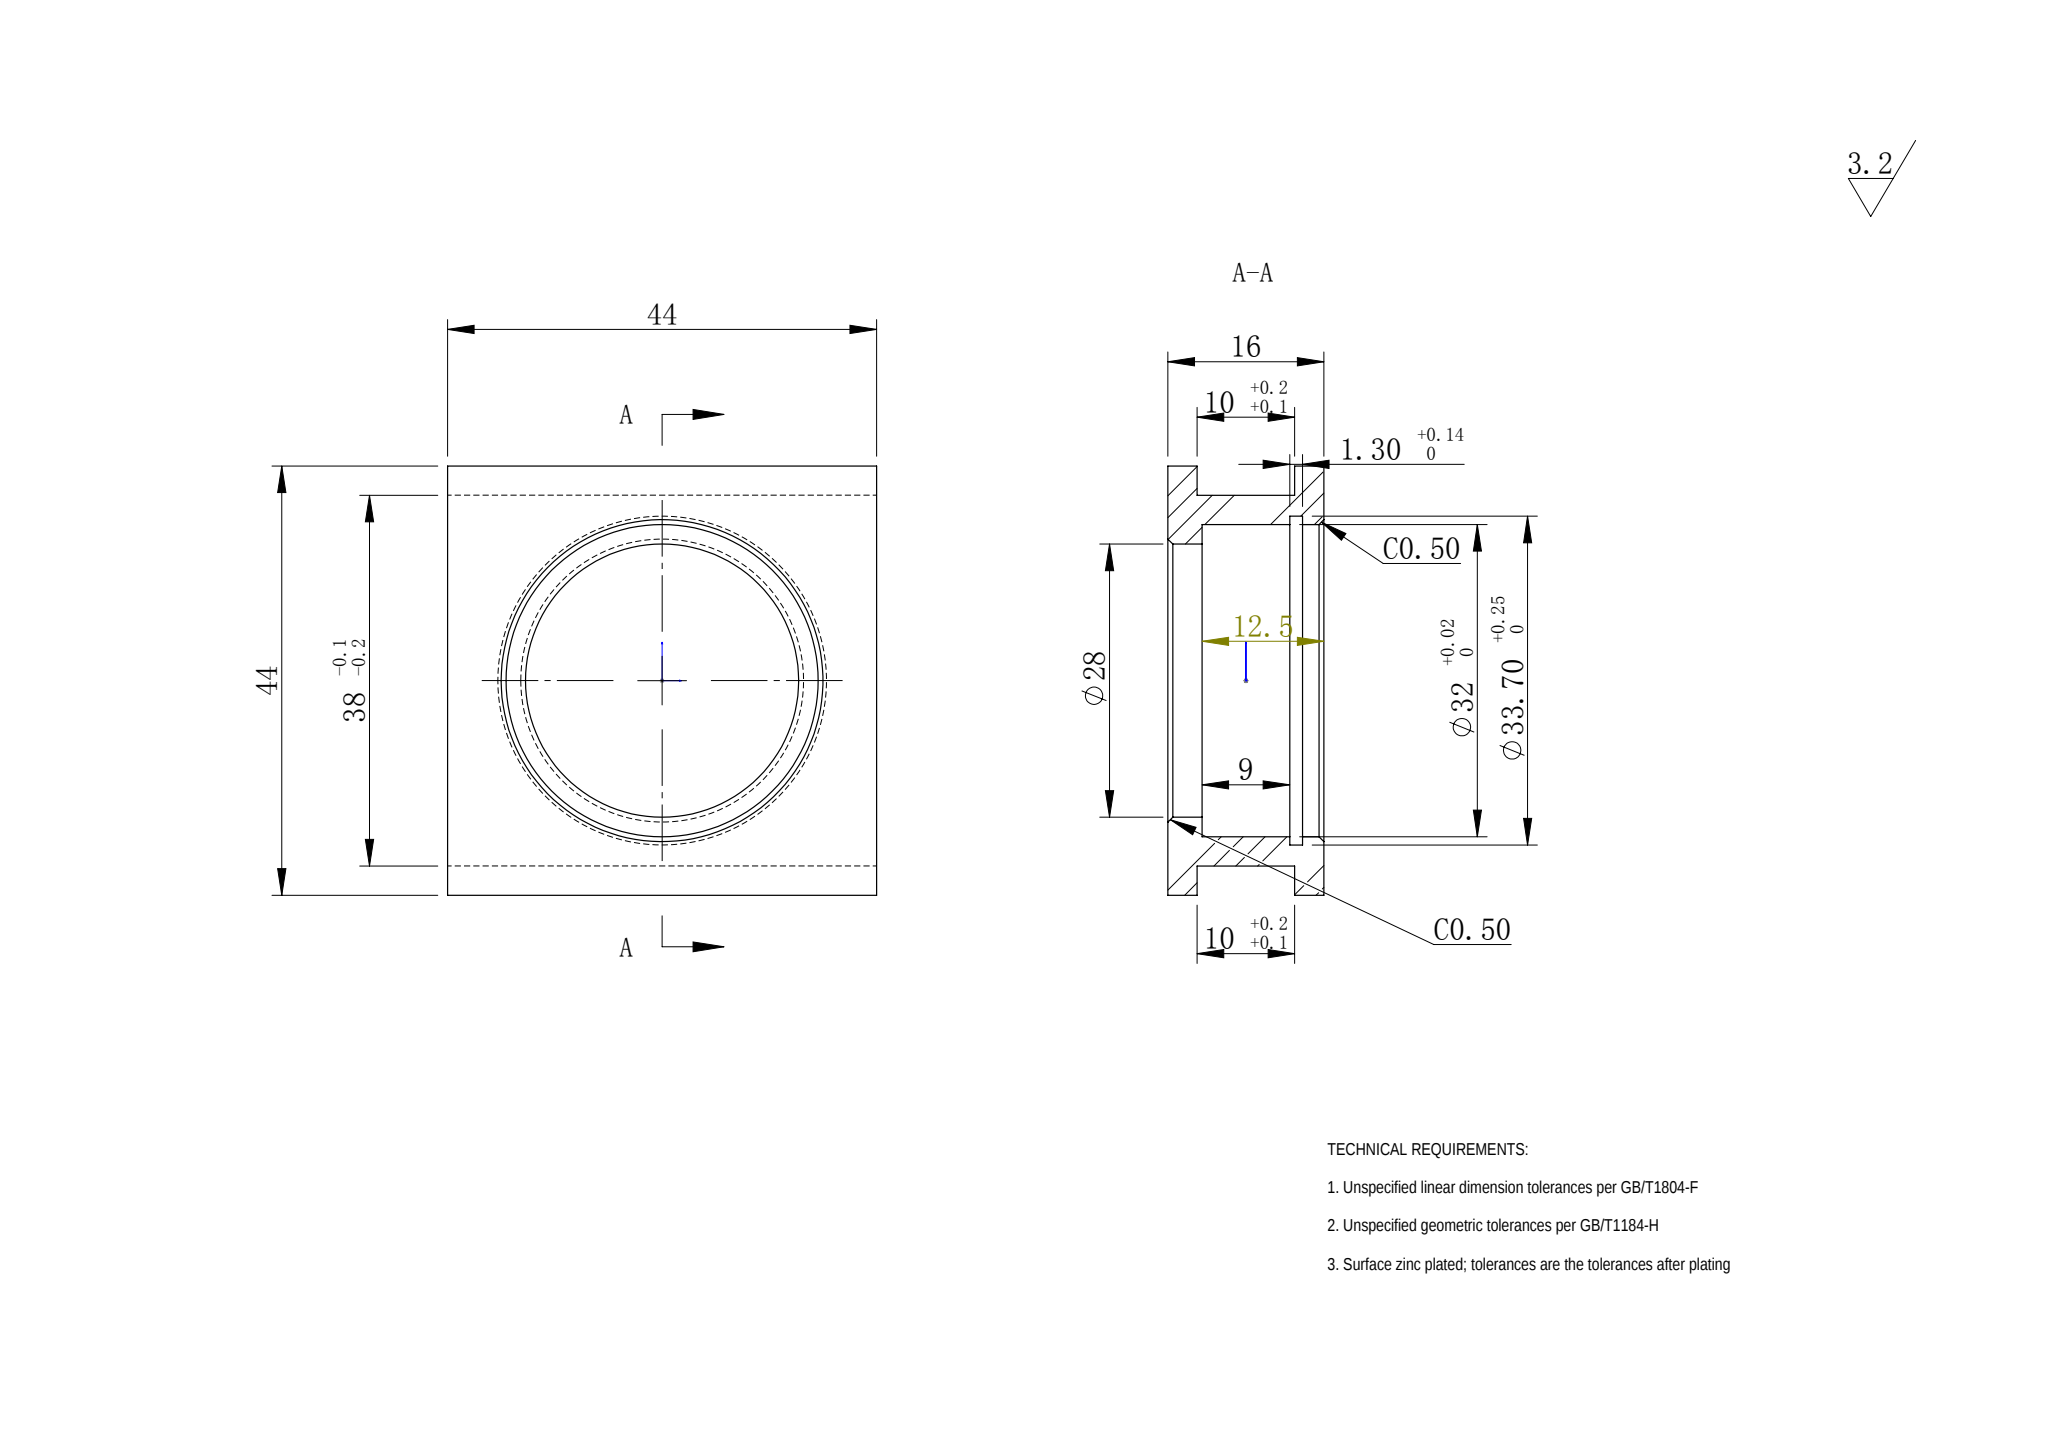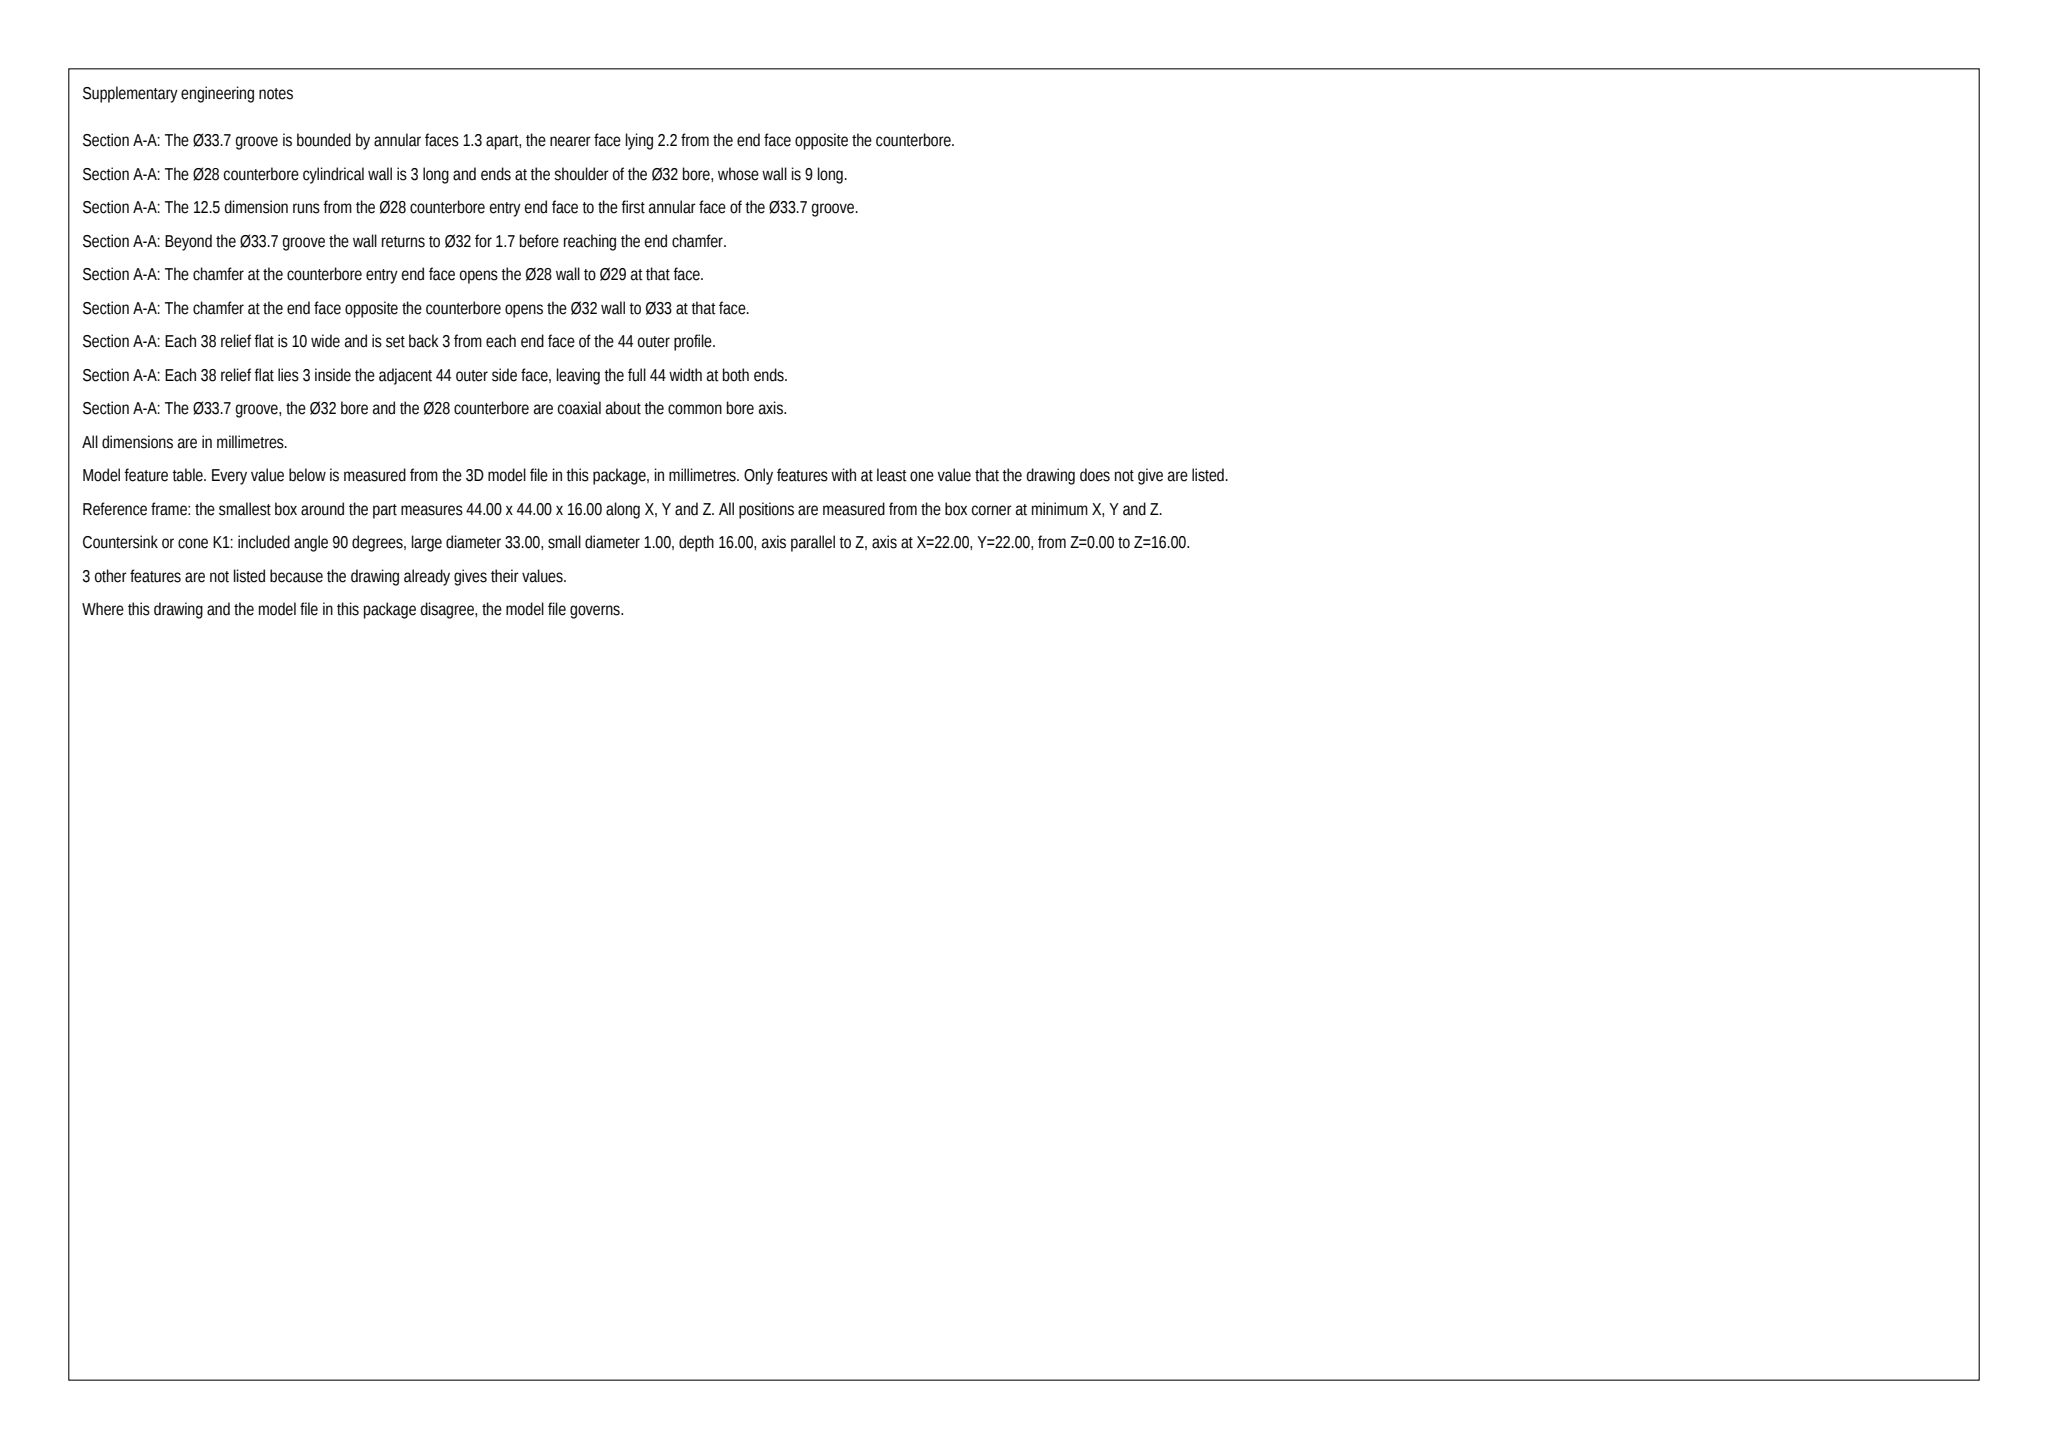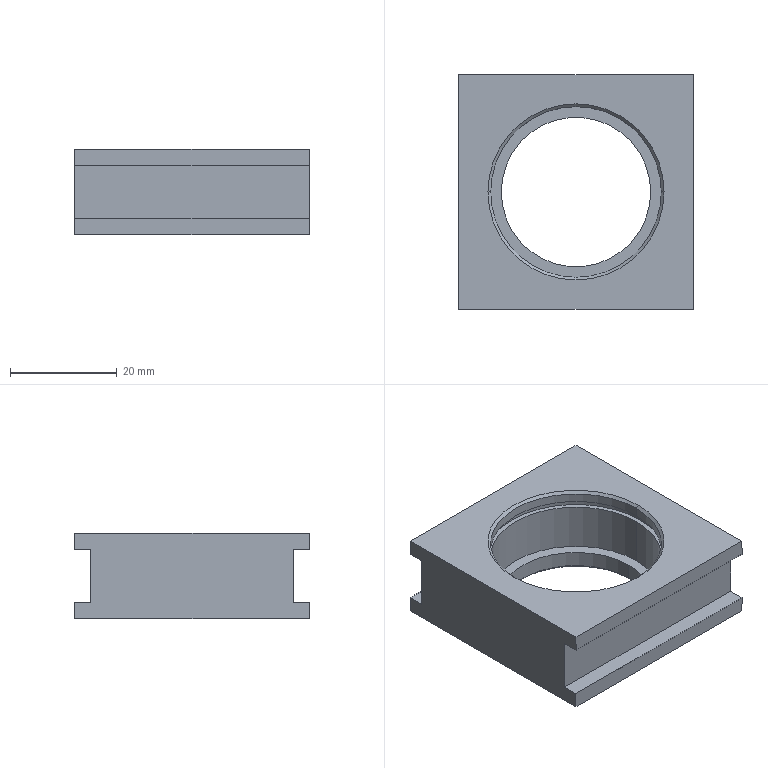Part | SolidWorks | mm | 1 solid | 29 faces | box 44 x 44 x 16 mm | volume 15990 mm3 | plane 17 | cylinder 8 | cone 4 | commonest cylinder face diameters 32 x4 33.7 x2 28 x2
build123d program:
from build123d import *

# Parameters (mm, degrees)
SKETCH1_W           = 44
SKETCH1_H           = 44
BOSS_EXTRUDE1_DEPTH = 8
SKETCH2_R           = 16
CUT_EXTRUDE1_DEPTH  = 12.5
SKETCH3_R           = 14
CUT_EXTRUDE2_DEPTH  = 34.53
SKETCH5_W           = 1.3
SKETCH5_H           = 0.85
SKETCH6_W           = 10
SKETCH6_H           = 3
CUT_EXTRUDE3_DEPTH  = 50.84
CHAMFER1_SIZE       = 0.5


with BuildPart() as part:
    # Sketch1 → Boss-Extrude1 (new, symmetric)
    with BuildSketch(Plane.XY):
        Rectangle(SKETCH1_W, SKETCH1_H)
    extrude(amount=BOSS_EXTRUDE1_DEPTH, both=True)

    # Sketch2 → Cut-Extrude1 (cut)
    with BuildSketch(Plane.XY.offset(8)):
        Circle(SKETCH2_R)
    extrude(amount=-CUT_EXTRUDE1_DEPTH, mode=Mode.SUBTRACT)

    # Sketch3 → Cut-Extrude2 (cut, through all)
    with BuildSketch(Plane.XY.offset(-4.5)):
        Circle(SKETCH3_R)
    extrude(amount=-CUT_EXTRUDE2_DEPTH, mode=Mode.SUBTRACT)

    # Sketch5 → Cut-Revolve1 (revolve, cut)
    with BuildSketch(Plane(origin=(0, 0, 0), x_dir=(0, 0, -1), z_dir=(1, 0, 0)), mode=Mode.PRIVATE) as cut_revolve1_sk:
        with Locations((-5.15, 16.425)):
            Rectangle(SKETCH5_W, SKETCH5_H)
    revolve(cut_revolve1_sk.sketch.rotate(Axis((0, 0, -9.603), (0, 0, 1)), 270), axis=Axis((0, 0, -9.603), (0, 0, 1)), mode=Mode.SUBTRACT)

    # Sketch6 → Cut-Extrude3 (cut, through all)
    with BuildSketch(Plane(origin=(22, 0, 0), x_dir=(0, 0, -1), z_dir=(1, 0, 0))):
        with Locations((0, 20.5)):
            Rectangle(SKETCH6_W, SKETCH6_H)
        with Locations((0, -20.5)):
            Rectangle(SKETCH6_W, SKETCH6_H)
    extrude(amount=-CUT_EXTRUDE3_DEPTH, mode=Mode.SUBTRACT)

    # Chamfer1
    chamfer1_edges = [part.edges().sort_by_distance(p)[0] for p in [
        (-16, 0, 8),
        (-14, 0, -8),
    ]]
    chamfer(chamfer1_edges, length=CHAMFER1_SIZE)


solid = part.part
STEP:
#1=CARTESIAN_POINT('',(-16.,0.,7.5));
#2=VERTEX_POINT('',#1);
#3=CARTESIAN_POINT('',(16.,0.,7.5));
#4=VERTEX_POINT('',#3);
#5=CARTESIAN_POINT('',(0.,0.,7.5));
#6=DIRECTION('',(0.,0.,1.));
#7=DIRECTION('',(-1.,0.,0.));
#8=AXIS2_PLACEMENT_3D('',#5,#6,#7);
#9=CIRCLE('',#8,16.);
#10=EDGE_CURVE('',#2,#4,#9,.T.);
#11=ORIENTED_EDGE('',*,*,#10,.F.);
#12=CARTESIAN_POINT('',(-16.5,0.,8.));
#13=VERTEX_POINT('',#12);
#14=CARTESIAN_POINT('',(-16.,0.,7.5));
#15=DIRECTION('',(-0.7071,0.,0.7071));
#16=VECTOR('',#15,1000.);
#17=LINE('',#14,#16);
#18=EDGE_CURVE('',#2,#13,#17,.T.);
#19=ORIENTED_EDGE('',*,*,#18,.T.);
#20=CARTESIAN_POINT('',(16.5,0.,8.));
#21=VERTEX_POINT('',#20);
#22=CARTESIAN_POINT('',(0.,0.,8.));
#23=DIRECTION('',(0.,0.,-1.));
#24=DIRECTION('',(-1.,0.,0.));
#25=AXIS2_PLACEMENT_3D('',#22,#23,#24);
#26=CIRCLE('',#25,16.5);
#27=EDGE_CURVE('',#21,#13,#26,.T.);
#28=ORIENTED_EDGE('',*,*,#27,.F.);
#29=CARTESIAN_POINT('',(16.,0.,7.5));
#30=DIRECTION('',(0.7071,0.,0.7071));
#31=VECTOR('',#30,1000.);
#32=LINE('',#29,#31);
#33=EDGE_CURVE('',#4,#21,#32,.T.);
#34=ORIENTED_EDGE('',*,*,#33,.F.);
#35=EDGE_LOOP('',(#11,#19,#28,#34));
#36=FACE_OUTER_BOUND('',#35,.T.);
#37=CARTESIAN_POINT('',(0.,0.,7.5));
#38=DIRECTION('',(0.,0.,1.));
#39=DIRECTION('',(1.,0.,0.));
#40=AXIS2_PLACEMENT_3D('',#37,#38,#39);
#41=CONICAL_SURFACE('',#40,16.,0.7854);
#42=ADVANCED_FACE('',(#36),#41,.F.);
#43=CARTESIAN_POINT('',(14.,0.,-7.5));
#44=VERTEX_POINT('',#43);
#45=CARTESIAN_POINT('',(-14.,0.,-7.5));
#46=VERTEX_POINT('',#45);
#47=CARTESIAN_POINT('',(0.,0.,-7.5));
#48=DIRECTION('',(0.,0.,-1.));
#49=DIRECTION('',(-1.,0.,0.));
#50=AXIS2_PLACEMENT_3D('',#47,#48,#49);
#51=CIRCLE('',#50,14.);
#52=EDGE_CURVE('',#44,#46,#51,.T.);
#53=ORIENTED_EDGE('',*,*,#52,.F.);
#54=CARTESIAN_POINT('',(14.5,0.,-8.));
#55=VERTEX_POINT('',#54);
#56=CARTESIAN_POINT('',(14.5,0.,-8.));
#57=DIRECTION('',(0.7071,0.,-0.7071));
#58=VECTOR('',#57,1000.);
#59=LINE('',#56,#58);
#60=EDGE_CURVE('',#44,#55,#59,.T.);
#61=ORIENTED_EDGE('',*,*,#60,.T.);
#62=CARTESIAN_POINT('',(-14.5,0.,-8.));
#63=VERTEX_POINT('',#62);
#64=CARTESIAN_POINT('',(0.,0.,-8.));
#65=DIRECTION('',(0.,0.,1.));
#66=DIRECTION('',(-1.,0.,0.));
#67=AXIS2_PLACEMENT_3D('',#64,#65,#66);
#68=CIRCLE('',#67,14.5);
#69=EDGE_CURVE('',#63,#55,#68,.T.);
#70=ORIENTED_EDGE('',*,*,#69,.F.);
#71=CARTESIAN_POINT('',(-14.5,0.,-8.));
#72=DIRECTION('',(-0.7071,0.,-0.7071));
#73=VECTOR('',#72,1000.);
#74=LINE('',#71,#73);
#75=EDGE_CURVE('',#46,#63,#74,.T.);
#76=ORIENTED_EDGE('',*,*,#75,.F.);
#77=EDGE_LOOP('',(#53,#61,#70,#76));
#78=FACE_OUTER_BOUND('',#77,.T.);
#79=CARTESIAN_POINT('',(0.,0.,-8.));
#80=DIRECTION('',(0.,0.,-1.));
#81=DIRECTION('',(-1.,0.,0.));
#82=AXIS2_PLACEMENT_3D('',#79,#80,#81);
#83=CONICAL_SURFACE('',#82,14.5,0.7854);
#84=ADVANCED_FACE('',(#78),#83,.F.);
#85=CARTESIAN_POINT('',(16.85,0.,5.8));
#86=VERTEX_POINT('',#85);
#87=CARTESIAN_POINT('',(-16.85,0.,5.8));
#88=VERTEX_POINT('',#87);
#89=CARTESIAN_POINT('',(0.,0.,5.8));
#90=DIRECTION('',(0.,0.,-1.));
#91=DIRECTION('',(-1.,0.,0.));
#92=AXIS2_PLACEMENT_3D('',#89,#90,#91);
#93=CIRCLE('',#92,16.85);
#94=EDGE_CURVE('',#86,#88,#93,.T.);
#95=ORIENTED_EDGE('',*,*,#94,.F.);
#96=CARTESIAN_POINT('',(16.85,0.,4.5));
#97=VERTEX_POINT('',#96);
#98=CARTESIAN_POINT('',(16.85,0.,-9.603));
#99=DIRECTION('',(0.,0.,-1.));
#100=VECTOR('',#99,1000.);
#101=LINE('',#98,#100);
#102=EDGE_CURVE('',#86,#97,#101,.T.);
#103=ORIENTED_EDGE('',*,*,#102,.T.);
#104=CARTESIAN_POINT('',(-16.85,0.,4.5));
#105=VERTEX_POINT('',#104);
#106=CARTESIAN_POINT('',(0.,0.,4.5));
#107=DIRECTION('',(0.,0.,-1.));
#108=DIRECTION('',(-1.,0.,0.));
#109=AXIS2_PLACEMENT_3D('',#106,#107,#108);
#110=CIRCLE('',#109,16.85);
#111=EDGE_CURVE('',#97,#105,#110,.T.);
#112=ORIENTED_EDGE('',*,*,#111,.T.);
#113=CARTESIAN_POINT('',(-16.85,0.,-9.603));
#114=DIRECTION('',(0.,0.,-1.));
#115=VECTOR('',#114,1000.);
#116=LINE('',#113,#115);
#117=EDGE_CURVE('',#88,#105,#116,.T.);
#118=ORIENTED_EDGE('',*,*,#117,.F.);
#119=EDGE_LOOP('',(#95,#103,#112,#118));
#120=FACE_OUTER_BOUND('',#119,.T.);
#121=CARTESIAN_POINT('',(0.,0.,-9.603));
#122=DIRECTION('',(0.,0.,-1.));
#123=DIRECTION('',(-1.,0.,0.));
#124=AXIS2_PLACEMENT_3D('',#121,#122,#123);
#125=CYLINDRICAL_SURFACE('',#124,16.85);
#126=ADVANCED_FACE('',(#120),#125,.F.);
#127=ORIENTED_EDGE('',*,*,#52,.T.);
#128=CARTESIAN_POINT('',(-14.,0.,-4.5));
#129=VERTEX_POINT('',#128);
#130=CARTESIAN_POINT('',(-14.,0.,-8.));
#131=DIRECTION('',(0.,0.,1.));
#132=VECTOR('',#131,1000.);
#133=LINE('',#130,#132);
#134=EDGE_CURVE('',#46,#129,#133,.T.);
#135=ORIENTED_EDGE('',*,*,#134,.T.);
#136=CARTESIAN_POINT('',(14.,0.,-4.5));
#137=VERTEX_POINT('',#136);
#138=CARTESIAN_POINT('',(0.,0.,-4.5));
#139=DIRECTION('',(0.,0.,1.));
#140=DIRECTION('',(1.,0.,0.));
#141=AXIS2_PLACEMENT_3D('',#138,#139,#140);
#142=CIRCLE('',#141,14.);
#143=EDGE_CURVE('',#129,#137,#142,.T.);
#144=ORIENTED_EDGE('',*,*,#143,.T.);
#145=CARTESIAN_POINT('',(14.,0.,-8.));
#146=DIRECTION('',(0.,0.,1.));
#147=VECTOR('',#146,1000.);
#148=LINE('',#145,#147);
#149=EDGE_CURVE('',#44,#137,#148,.T.);
#150=ORIENTED_EDGE('',*,*,#149,.F.);
#151=EDGE_LOOP('',(#127,#135,#144,#150));
#152=FACE_OUTER_BOUND('',#151,.T.);
#153=CARTESIAN_POINT('',(0.,0.,-8.));
#154=DIRECTION('',(0.,0.,1.));
#155=DIRECTION('',(1.,0.,0.));
#156=AXIS2_PLACEMENT_3D('',#153,#154,#155);
#157=CYLINDRICAL_SURFACE('',#156,14.);
#158=ADVANCED_FACE('',(#152),#157,.F.);
#159=CARTESIAN_POINT('',(16.,0.,5.8));
#160=VERTEX_POINT('',#159);
#161=CARTESIAN_POINT('',(-16.,0.,5.8));
#162=VERTEX_POINT('',#161);
#163=CARTESIAN_POINT('',(0.,0.,5.8));
#164=DIRECTION('',(0.,0.,-1.));
#165=DIRECTION('',(-1.,0.,0.));
#166=AXIS2_PLACEMENT_3D('',#163,#164,#165);
#167=CIRCLE('',#166,16.);
#168=EDGE_CURVE('',#160,#162,#167,.T.);
#169=ORIENTED_EDGE('',*,*,#168,.T.);
#170=CARTESIAN_POINT('',(-16.,0.,-4.5));
#171=DIRECTION('',(0.,0.,1.));
#172=VECTOR('',#171,1000.);
#173=LINE('',#170,#172);
#174=EDGE_CURVE('',#162,#2,#173,.T.);
#175=ORIENTED_EDGE('',*,*,#174,.T.);
#176=ORIENTED_EDGE('',*,*,#10,.T.);
#177=CARTESIAN_POINT('',(16.,0.,-4.5));
#178=DIRECTION('',(0.,0.,1.));
#179=VECTOR('',#178,1000.);
#180=LINE('',#177,#179);
#181=EDGE_CURVE('',#160,#4,#180,.T.);
#182=ORIENTED_EDGE('',*,*,#181,.F.);
#183=EDGE_LOOP('',(#169,#175,#176,#182));
#184=FACE_OUTER_BOUND('',#183,.T.);
#185=CARTESIAN_POINT('',(0.,0.,-4.5));
#186=DIRECTION('',(0.,0.,1.));
#187=DIRECTION('',(1.,0.,0.));
#188=AXIS2_PLACEMENT_3D('',#185,#186,#187);
#189=CYLINDRICAL_SURFACE('',#188,16.);
#190=ADVANCED_FACE('',(#184),#189,.F.);
#191=CARTESIAN_POINT('',(-16.,0.,-4.5));
#192=VERTEX_POINT('',#191);
#193=CARTESIAN_POINT('',(16.,0.,-4.5));
#194=VERTEX_POINT('',#193);
#195=CARTESIAN_POINT('',(0.,0.,-4.5));
#196=DIRECTION('',(0.,0.,1.));
#197=DIRECTION('',(1.,0.,0.));
#198=AXIS2_PLACEMENT_3D('',#195,#196,#197);
#199=CIRCLE('',#198,16.);
#200=EDGE_CURVE('',#192,#194,#199,.T.);
#201=ORIENTED_EDGE('',*,*,#200,.F.);
#202=CARTESIAN_POINT('',(-16.,0.,4.5));
#203=VERTEX_POINT('',#202);
#204=CARTESIAN_POINT('',(-16.,0.,-4.5));
#205=DIRECTION('',(0.,0.,1.));
#206=VECTOR('',#205,1000.);
#207=LINE('',#204,#206);
#208=EDGE_CURVE('',#192,#203,#207,.T.);
#209=ORIENTED_EDGE('',*,*,#208,.T.);
#210=CARTESIAN_POINT('',(16.,0.,4.5));
#211=VERTEX_POINT('',#210);
#212=CARTESIAN_POINT('',(0.,0.,4.5));
#213=DIRECTION('',(0.,0.,-1.));
#214=DIRECTION('',(-1.,0.,0.));
#215=AXIS2_PLACEMENT_3D('',#212,#213,#214);
#216=CIRCLE('',#215,16.);
#217=EDGE_CURVE('',#211,#203,#216,.T.);
#218=ORIENTED_EDGE('',*,*,#217,.F.);
#219=CARTESIAN_POINT('',(16.,0.,-4.5));
#220=DIRECTION('',(0.,0.,1.));
#221=VECTOR('',#220,1000.);
#222=LINE('',#219,#221);
#223=EDGE_CURVE('',#194,#211,#222,.T.);
#224=ORIENTED_EDGE('',*,*,#223,.F.);
#225=EDGE_LOOP('',(#201,#209,#218,#224));
#226=FACE_OUTER_BOUND('',#225,.T.);
#227=CARTESIAN_POINT('',(0.,0.,-4.5));
#228=DIRECTION('',(0.,0.,1.));
#229=DIRECTION('',(1.,0.,0.));
#230=AXIS2_PLACEMENT_3D('',#227,#228,#229);
#231=CYLINDRICAL_SURFACE('',#230,16.);
#232=ADVANCED_FACE('',(#226),#231,.F.);
#233=CARTESIAN_POINT('',(-22.,-22.,8.));
#234=VERTEX_POINT('',#233);
#235=CARTESIAN_POINT('',(-22.,-22.,5.));
#236=VERTEX_POINT('',#235);
#237=CARTESIAN_POINT('',(-22.,-22.,8.));
#238=DIRECTION('',(0.,0.,-1.));
#239=VECTOR('',#238,1000.);
#240=LINE('',#237,#239);
#241=EDGE_CURVE('',#234,#236,#240,.T.);
#242=ORIENTED_EDGE('',*,*,#241,.T.);
#243=CARTESIAN_POINT('',(22.,-22.,5.));
#244=VERTEX_POINT('',#243);
#245=CARTESIAN_POINT('',(-22.,-22.,5.));
#246=DIRECTION('',(1.,0.,0.));
#247=VECTOR('',#246,1000.);
#248=LINE('',#245,#247);
#249=EDGE_CURVE('',#236,#244,#248,.T.);
#250=ORIENTED_EDGE('',*,*,#249,.T.);
#251=CARTESIAN_POINT('',(22.,-22.,8.));
#252=VERTEX_POINT('',#251);
#253=CARTESIAN_POINT('',(22.,-22.,8.));
#254=DIRECTION('',(0.,0.,-1.));
#255=VECTOR('',#254,1000.);
#256=LINE('',#253,#255);
#257=EDGE_CURVE('',#252,#244,#256,.T.);
#258=ORIENTED_EDGE('',*,*,#257,.F.);
#259=CARTESIAN_POINT('',(-22.,-22.,8.));
#260=DIRECTION('',(1.,0.,0.));
#261=VECTOR('',#260,1000.);
#262=LINE('',#259,#261);
#263=EDGE_CURVE('',#234,#252,#262,.T.);
#264=ORIENTED_EDGE('',*,*,#263,.F.);
#265=EDGE_LOOP('',(#242,#250,#258,#264));
#266=FACE_OUTER_BOUND('',#265,.T.);
#267=CARTESIAN_POINT('',(-22.,-22.,8.));
#268=DIRECTION('',(0.,1.,0.));
#269=DIRECTION('',(0.,0.,1.));
#270=AXIS2_PLACEMENT_3D('',#267,#268,#269);
#271=PLANE('',#270);
#272=ADVANCED_FACE('',(#266),#271,.F.);
#273=CARTESIAN_POINT('',(22.,22.,8.));
#274=VERTEX_POINT('',#273);
#275=CARTESIAN_POINT('',(22.,22.,5.));
#276=VERTEX_POINT('',#275);
#277=CARTESIAN_POINT('',(22.,22.,8.));
#278=DIRECTION('',(0.,0.,-1.));
#279=VECTOR('',#278,1000.);
#280=LINE('',#277,#279);
#281=EDGE_CURVE('',#274,#276,#280,.T.);
#282=ORIENTED_EDGE('',*,*,#281,.T.);
#283=CARTESIAN_POINT('',(-22.,22.,5.));
#284=VERTEX_POINT('',#283);
#285=CARTESIAN_POINT('',(-22.,22.,5.));
#286=DIRECTION('',(1.,0.,0.));
#287=VECTOR('',#286,1000.);
#288=LINE('',#285,#287);
#289=EDGE_CURVE('',#284,#276,#288,.T.);
#290=ORIENTED_EDGE('',*,*,#289,.F.);
#291=CARTESIAN_POINT('',(-22.,22.,8.));
#292=VERTEX_POINT('',#291);
#293=CARTESIAN_POINT('',(-22.,22.,8.));
#294=DIRECTION('',(0.,0.,-1.));
#295=VECTOR('',#294,1000.);
#296=LINE('',#293,#295);
#297=EDGE_CURVE('',#292,#284,#296,.T.);
#298=ORIENTED_EDGE('',*,*,#297,.F.);
#299=CARTESIAN_POINT('',(-22.,22.,8.));
#300=DIRECTION('',(-1.,0.,0.));
#301=VECTOR('',#300,1000.);
#302=LINE('',#299,#301);
#303=EDGE_CURVE('',#274,#292,#302,.T.);
#304=ORIENTED_EDGE('',*,*,#303,.F.);
#305=EDGE_LOOP('',(#282,#290,#298,#304));
#306=FACE_OUTER_BOUND('',#305,.T.);
#307=CARTESIAN_POINT('',(-22.,22.,8.));
#308=DIRECTION('',(0.,-1.,0.));
#309=DIRECTION('',(0.,0.,-1.));
#310=AXIS2_PLACEMENT_3D('',#307,#308,#309);
#311=PLANE('',#310);
#312=ADVANCED_FACE('',(#306),#311,.F.);
#313=ORIENTED_EDGE('',*,*,#208,.F.);
#314=CARTESIAN_POINT('',(0.,0.,-4.5));
#315=DIRECTION('',(0.,0.,1.));
#316=DIRECTION('',(1.,0.,0.));
#317=AXIS2_PLACEMENT_3D('',#314,#315,#316);
#318=CIRCLE('',#317,16.);
#319=EDGE_CURVE('',#194,#192,#318,.T.);
#320=ORIENTED_EDGE('',*,*,#319,.F.);
#321=ORIENTED_EDGE('',*,*,#223,.T.);
#322=CARTESIAN_POINT('',(0.,0.,4.5));
#323=DIRECTION('',(0.,0.,-1.));
#324=DIRECTION('',(-1.,0.,0.));
#325=AXIS2_PLACEMENT_3D('',#322,#323,#324);
#326=CIRCLE('',#325,16.);
#327=EDGE_CURVE('',#203,#211,#326,.T.);
#328=ORIENTED_EDGE('',*,*,#327,.F.);
#329=EDGE_LOOP('',(#313,#320,#321,#328));
#330=FACE_OUTER_BOUND('',#329,.T.);
#331=CARTESIAN_POINT('',(0.,0.,-4.5));
#332=DIRECTION('',(0.,0.,1.));
#333=DIRECTION('',(1.,0.,0.));
#334=AXIS2_PLACEMENT_3D('',#331,#332,#333);
#335=CYLINDRICAL_SURFACE('',#334,16.);
#336=ADVANCED_FACE('',(#330),#335,.F.);
#337=ORIENTED_EDGE('',*,*,#257,.T.);
#338=CARTESIAN_POINT('',(22.,-19.,5.));
#339=VERTEX_POINT('',#338);
#340=CARTESIAN_POINT('',(22.,-22.,5.));
#341=DIRECTION('',(0.,-1.,-0.));
#342=VECTOR('',#341,1000.);
#343=LINE('',#340,#342);
#344=EDGE_CURVE('',#339,#244,#343,.T.);
#345=ORIENTED_EDGE('',*,*,#344,.F.);
#346=CARTESIAN_POINT('',(22.,-19.,-5.));
#347=VERTEX_POINT('',#346);
#348=CARTESIAN_POINT('',(22.,-19.,5.));
#349=DIRECTION('',(0.,0.,1.));
#350=VECTOR('',#349,1000.);
#351=LINE('',#348,#350);
#352=EDGE_CURVE('',#347,#339,#351,.T.);
#353=ORIENTED_EDGE('',*,*,#352,.F.);
#354=CARTESIAN_POINT('',(22.,-22.,-5.));
#355=VERTEX_POINT('',#354);
#356=CARTESIAN_POINT('',(22.,-22.,-5.));
#357=DIRECTION('',(0.,1.,-0.));
#358=VECTOR('',#357,1000.);
#359=LINE('',#356,#358);
#360=EDGE_CURVE('',#355,#347,#359,.T.);
#361=ORIENTED_EDGE('',*,*,#360,.F.);
#362=CARTESIAN_POINT('',(22.,-22.,-8.));
#363=VERTEX_POINT('',#362);
#364=CARTESIAN_POINT('',(22.,-22.,8.));
#365=DIRECTION('',(0.,0.,-1.));
#366=VECTOR('',#365,1000.);
#367=LINE('',#364,#366);
#368=EDGE_CURVE('',#355,#363,#367,.T.);
#369=ORIENTED_EDGE('',*,*,#368,.T.);
#370=CARTESIAN_POINT('',(22.,22.,-8.));
#371=VERTEX_POINT('',#370);
#372=CARTESIAN_POINT('',(22.,-22.,-8.));
#373=DIRECTION('',(0.,1.,0.));
#374=VECTOR('',#373,1000.);
#375=LINE('',#372,#374);
#376=EDGE_CURVE('',#363,#371,#375,.T.);
#377=ORIENTED_EDGE('',*,*,#376,.T.);
#378=CARTESIAN_POINT('',(22.,22.,-5.));
#379=VERTEX_POINT('',#378);
#380=CARTESIAN_POINT('',(22.,22.,8.));
#381=DIRECTION('',(0.,0.,-1.));
#382=VECTOR('',#381,1000.);
#383=LINE('',#380,#382);
#384=EDGE_CURVE('',#379,#371,#383,.T.);
#385=ORIENTED_EDGE('',*,*,#384,.F.);
#386=CARTESIAN_POINT('',(22.,19.,-5.));
#387=VERTEX_POINT('',#386);
#388=CARTESIAN_POINT('',(22.,22.,-5.));
#389=DIRECTION('',(0.,1.,0.));
#390=VECTOR('',#389,1000.);
#391=LINE('',#388,#390);
#392=EDGE_CURVE('',#387,#379,#391,.T.);
#393=ORIENTED_EDGE('',*,*,#392,.F.);
#394=CARTESIAN_POINT('',(22.,19.,5.));
#395=VERTEX_POINT('',#394);
#396=CARTESIAN_POINT('',(22.,19.,5.));
#397=DIRECTION('',(0.,0.,-1.));
#398=VECTOR('',#397,1000.);
#399=LINE('',#396,#398);
#400=EDGE_CURVE('',#395,#387,#399,.T.);
#401=ORIENTED_EDGE('',*,*,#400,.F.);
#402=CARTESIAN_POINT('',(22.,22.,5.));
#403=DIRECTION('',(0.,-1.,0.));
#404=VECTOR('',#403,1000.);
#405=LINE('',#402,#404);
#406=EDGE_CURVE('',#276,#395,#405,.T.);
#407=ORIENTED_EDGE('',*,*,#406,.F.);
#408=ORIENTED_EDGE('',*,*,#281,.F.);
#409=CARTESIAN_POINT('',(22.,-22.,8.));
#410=DIRECTION('',(0.,1.,0.));
#411=VECTOR('',#410,1000.);
#412=LINE('',#409,#411);
#413=EDGE_CURVE('',#252,#274,#412,.T.);
#414=ORIENTED_EDGE('',*,*,#413,.F.);
#415=EDGE_LOOP('',(#337,#345,#353,#361,#369,#377,#385,#393,#401,#407,#408,#414));
#416=FACE_OUTER_BOUND('',#415,.T.);
#417=CARTESIAN_POINT('',(22.,-22.,8.));
#418=DIRECTION('',(-1.,0.,0.));
#419=DIRECTION('',(0.,0.,1.));
#420=AXIS2_PLACEMENT_3D('',#417,#418,#419);
#421=PLANE('',#420);
#422=ADVANCED_FACE('',(#416),#421,.F.);
#423=CARTESIAN_POINT('',(-22.,22.,-5.));
#424=VERTEX_POINT('',#423);
#425=CARTESIAN_POINT('',(-22.,22.,-8.));
#426=VERTEX_POINT('',#425);
#427=CARTESIAN_POINT('',(-22.,22.,8.));
#428=DIRECTION('',(0.,0.,-1.));
#429=VECTOR('',#428,1000.);
#430=LINE('',#427,#429);
#431=EDGE_CURVE('',#424,#426,#430,.T.);
#432=ORIENTED_EDGE('',*,*,#431,.F.);
#433=CARTESIAN_POINT('',(-22.,22.,-5.));
#434=DIRECTION('',(1.,0.,0.));
#435=VECTOR('',#434,1000.);
#436=LINE('',#433,#435);
#437=EDGE_CURVE('',#424,#379,#436,.T.);
#438=ORIENTED_EDGE('',*,*,#437,.T.);
#439=ORIENTED_EDGE('',*,*,#384,.T.);
#440=CARTESIAN_POINT('',(-22.,22.,-8.));
#441=DIRECTION('',(-1.,0.,0.));
#442=VECTOR('',#441,1000.);
#443=LINE('',#440,#442);
#444=EDGE_CURVE('',#371,#426,#443,.T.);
#445=ORIENTED_EDGE('',*,*,#444,.T.);
#446=EDGE_LOOP('',(#432,#438,#439,#445));
#447=FACE_OUTER_BOUND('',#446,.T.);
#448=CARTESIAN_POINT('',(-22.,22.,8.));
#449=DIRECTION('',(0.,-1.,0.));
#450=DIRECTION('',(0.,0.,-1.));
#451=AXIS2_PLACEMENT_3D('',#448,#449,#450);
#452=PLANE('',#451);
#453=ADVANCED_FACE('',(#447),#452,.F.);
#454=CARTESIAN_POINT('',(-22.,-19.,-5.));
#455=VERTEX_POINT('',#454);
#456=CARTESIAN_POINT('',(-22.,-19.,5.));
#457=VERTEX_POINT('',#456);
#458=CARTESIAN_POINT('',(-22.,-19.,5.));
#459=DIRECTION('',(0.,0.,1.));
#460=VECTOR('',#459,1000.);
#461=LINE('',#458,#460);
#462=EDGE_CURVE('',#455,#457,#461,.T.);
#463=ORIENTED_EDGE('',*,*,#462,.T.);
#464=CARTESIAN_POINT('',(-22.,-22.,5.));
#465=DIRECTION('',(0.,-1.,-0.));
#466=VECTOR('',#465,1000.);
#467=LINE('',#464,#466);
#468=EDGE_CURVE('',#457,#236,#467,.T.);
#469=ORIENTED_EDGE('',*,*,#468,.T.);
#470=ORIENTED_EDGE('',*,*,#241,.F.);
#471=CARTESIAN_POINT('',(-22.,-22.,8.));
#472=DIRECTION('',(0.,-1.,0.));
#473=VECTOR('',#472,1000.);
#474=LINE('',#471,#473);
#475=EDGE_CURVE('',#292,#234,#474,.T.);
#476=ORIENTED_EDGE('',*,*,#475,.F.);
#477=ORIENTED_EDGE('',*,*,#297,.T.);
#478=CARTESIAN_POINT('',(-22.,19.,5.));
#479=VERTEX_POINT('',#478);
#480=CARTESIAN_POINT('',(-22.,22.,5.));
#481=DIRECTION('',(0.,-1.,0.));
#482=VECTOR('',#481,1000.);
#483=LINE('',#480,#482);
#484=EDGE_CURVE('',#284,#479,#483,.T.);
#485=ORIENTED_EDGE('',*,*,#484,.T.);
#486=CARTESIAN_POINT('',(-22.,19.,-5.));
#487=VERTEX_POINT('',#486);
#488=CARTESIAN_POINT('',(-22.,19.,5.));
#489=DIRECTION('',(0.,0.,-1.));
#490=VECTOR('',#489,1000.);
#491=LINE('',#488,#490);
#492=EDGE_CURVE('',#479,#487,#491,.T.);
#493=ORIENTED_EDGE('',*,*,#492,.T.);
#494=CARTESIAN_POINT('',(-22.,22.,-5.));
#495=DIRECTION('',(0.,1.,0.));
#496=VECTOR('',#495,1000.);
#497=LINE('',#494,#496);
#498=EDGE_CURVE('',#487,#424,#497,.T.);
#499=ORIENTED_EDGE('',*,*,#498,.T.);
#500=ORIENTED_EDGE('',*,*,#431,.T.);
#501=CARTESIAN_POINT('',(-22.,-22.,-8.));
#502=VERTEX_POINT('',#501);
#503=CARTESIAN_POINT('',(-22.,-22.,-8.));
#504=DIRECTION('',(0.,-1.,0.));
#505=VECTOR('',#504,1000.);
#506=LINE('',#503,#505);
#507=EDGE_CURVE('',#426,#502,#506,.T.);
#508=ORIENTED_EDGE('',*,*,#507,.T.);
#509=CARTESIAN_POINT('',(-22.,-22.,-5.));
#510=VERTEX_POINT('',#509);
#511=CARTESIAN_POINT('',(-22.,-22.,8.));
#512=DIRECTION('',(0.,0.,-1.));
#513=VECTOR('',#512,1000.);
#514=LINE('',#511,#513);
#515=EDGE_CURVE('',#510,#502,#514,.T.);
#516=ORIENTED_EDGE('',*,*,#515,.F.);
#517=CARTESIAN_POINT('',(-22.,-22.,-5.));
#518=DIRECTION('',(0.,1.,-0.));
#519=VECTOR('',#518,1000.);
#520=LINE('',#517,#519);
#521=EDGE_CURVE('',#510,#455,#520,.T.);
#522=ORIENTED_EDGE('',*,*,#521,.T.);
#523=EDGE_LOOP('',(#463,#469,#470,#476,#477,#485,#493,#499,#500,#508,#516,#522));
#524=FACE_OUTER_BOUND('',#523,.T.);
#525=CARTESIAN_POINT('',(-22.,-22.,8.));
#526=DIRECTION('',(1.,0.,0.));
#527=DIRECTION('',(0.,0.,-1.));
#528=AXIS2_PLACEMENT_3D('',#525,#526,#527);
#529=PLANE('',#528);
#530=ADVANCED_FACE('',(#524),#529,.F.);
#531=ORIENTED_EDGE('',*,*,#368,.F.);
#532=CARTESIAN_POINT('',(-22.,-22.,-5.));
#533=DIRECTION('',(1.,0.,0.));
#534=VECTOR('',#533,1000.);
#535=LINE('',#532,#534);
#536=EDGE_CURVE('',#510,#355,#535,.T.);
#537=ORIENTED_EDGE('',*,*,#536,.F.);
#538=ORIENTED_EDGE('',*,*,#515,.T.);
#539=CARTESIAN_POINT('',(-22.,-22.,-8.));
#540=DIRECTION('',(1.,0.,0.));
#541=VECTOR('',#540,1000.);
#542=LINE('',#539,#541);
#543=EDGE_CURVE('',#502,#363,#542,.T.);
#544=ORIENTED_EDGE('',*,*,#543,.T.);
#545=EDGE_LOOP('',(#531,#537,#538,#544));
#546=FACE_OUTER_BOUND('',#545,.T.);
#547=CARTESIAN_POINT('',(-22.,-22.,8.));
#548=DIRECTION('',(0.,1.,0.));
#549=DIRECTION('',(0.,0.,1.));
#550=AXIS2_PLACEMENT_3D('',#547,#548,#549);
#551=PLANE('',#550);
#552=ADVANCED_FACE('',(#546),#551,.F.);
#553=ORIENTED_EDGE('',*,*,#27,.T.);
#554=CARTESIAN_POINT('',(0.,0.,8.));
#555=DIRECTION('',(0.,0.,-1.));
#556=DIRECTION('',(-1.,0.,0.));
#557=AXIS2_PLACEMENT_3D('',#554,#555,#556);
#558=CIRCLE('',#557,16.5);
#559=EDGE_CURVE('',#13,#21,#558,.T.);
#560=ORIENTED_EDGE('',*,*,#559,.T.);
#561=EDGE_LOOP('',(#553,#560));
#562=FACE_BOUND('',#561,.T.);
#563=ORIENTED_EDGE('',*,*,#413,.T.);
#564=ORIENTED_EDGE('',*,*,#303,.T.);
#565=ORIENTED_EDGE('',*,*,#475,.T.);
#566=ORIENTED_EDGE('',*,*,#263,.T.);
#567=EDGE_LOOP('',(#563,#564,#565,#566));
#568=FACE_OUTER_BOUND('',#567,.T.);
#569=CARTESIAN_POINT('',(0.,0.,8.));
#570=DIRECTION('',(0.,0.,-1.));
#571=DIRECTION('',(-1.,0.,0.));
#572=AXIS2_PLACEMENT_3D('',#569,#570,#571);
#573=PLANE('',#572);
#574=ADVANCED_FACE('',(#562,#568),#573,.F.);
#575=ORIENTED_EDGE('',*,*,#69,.T.);
#576=CARTESIAN_POINT('',(0.,0.,-8.));
#577=DIRECTION('',(0.,0.,1.));
#578=DIRECTION('',(-1.,0.,0.));
#579=AXIS2_PLACEMENT_3D('',#576,#577,#578);
#580=CIRCLE('',#579,14.5);
#581=EDGE_CURVE('',#55,#63,#580,.T.);
#582=ORIENTED_EDGE('',*,*,#581,.T.);
#583=EDGE_LOOP('',(#575,#582));
#584=FACE_BOUND('',#583,.T.);
#585=ORIENTED_EDGE('',*,*,#376,.F.);
#586=ORIENTED_EDGE('',*,*,#543,.F.);
#587=ORIENTED_EDGE('',*,*,#507,.F.);
#588=ORIENTED_EDGE('',*,*,#444,.F.);
#589=EDGE_LOOP('',(#585,#586,#587,#588));
#590=FACE_OUTER_BOUND('',#589,.T.);
#591=CARTESIAN_POINT('',(0.,0.,-8.));
#592=DIRECTION('',(0.,0.,-1.));
#593=DIRECTION('',(-1.,0.,0.));
#594=AXIS2_PLACEMENT_3D('',#591,#592,#593);
#595=PLANE('',#594);
#596=ADVANCED_FACE('',(#584,#590),#595,.T.);
#597=ORIENTED_EDGE('',*,*,#174,.F.);
#598=CARTESIAN_POINT('',(0.,0.,5.8));
#599=DIRECTION('',(0.,0.,-1.));
#600=DIRECTION('',(-1.,0.,0.));
#601=AXIS2_PLACEMENT_3D('',#598,#599,#600);
#602=CIRCLE('',#601,16.);
#603=EDGE_CURVE('',#162,#160,#602,.T.);
#604=ORIENTED_EDGE('',*,*,#603,.T.);
#605=ORIENTED_EDGE('',*,*,#181,.T.);
#606=CARTESIAN_POINT('',(0.,0.,7.5));
#607=DIRECTION('',(0.,0.,1.));
#608=DIRECTION('',(-1.,0.,0.));
#609=AXIS2_PLACEMENT_3D('',#606,#607,#608);
#610=CIRCLE('',#609,16.);
#611=EDGE_CURVE('',#4,#2,#610,.T.);
#612=ORIENTED_EDGE('',*,*,#611,.T.);
#613=EDGE_LOOP('',(#597,#604,#605,#612));
#614=FACE_OUTER_BOUND('',#613,.T.);
#615=CARTESIAN_POINT('',(0.,0.,-4.5));
#616=DIRECTION('',(0.,0.,1.));
#617=DIRECTION('',(1.,0.,0.));
#618=AXIS2_PLACEMENT_3D('',#615,#616,#617);
#619=CYLINDRICAL_SURFACE('',#618,16.);
#620=ADVANCED_FACE('',(#614),#619,.F.);
#621=CARTESIAN_POINT('',(0.,0.,-4.5));
#622=DIRECTION('',(0.,0.,1.));
#623=DIRECTION('',(1.,0.,0.));
#624=AXIS2_PLACEMENT_3D('',#621,#622,#623);
#625=CIRCLE('',#624,14.);
#626=EDGE_CURVE('',#137,#129,#625,.T.);
#627=ORIENTED_EDGE('',*,*,#626,.F.);
#628=ORIENTED_EDGE('',*,*,#143,.F.);
#629=EDGE_LOOP('',(#627,#628));
#630=FACE_BOUND('',#629,.T.);
#631=ORIENTED_EDGE('',*,*,#319,.T.);
#632=ORIENTED_EDGE('',*,*,#200,.T.);
#633=EDGE_LOOP('',(#631,#632));
#634=FACE_OUTER_BOUND('',#633,.T.);
#635=CARTESIAN_POINT('',(0.,0.,-4.5));
#636=DIRECTION('',(0.,0.,1.));
#637=DIRECTION('',(1.,0.,0.));
#638=AXIS2_PLACEMENT_3D('',#635,#636,#637);
#639=PLANE('',#638);
#640=ADVANCED_FACE('',(#630,#634),#639,.T.);
#641=ORIENTED_EDGE('',*,*,#134,.F.);
#642=CARTESIAN_POINT('',(0.,0.,-7.5));
#643=DIRECTION('',(0.,0.,-1.));
#644=DIRECTION('',(-1.,0.,0.));
#645=AXIS2_PLACEMENT_3D('',#642,#643,#644);
#646=CIRCLE('',#645,14.);
#647=EDGE_CURVE('',#46,#44,#646,.T.);
#648=ORIENTED_EDGE('',*,*,#647,.T.);
#649=ORIENTED_EDGE('',*,*,#149,.T.);
#650=ORIENTED_EDGE('',*,*,#626,.T.);
#651=EDGE_LOOP('',(#641,#648,#649,#650));
#652=FACE_OUTER_BOUND('',#651,.T.);
#653=CARTESIAN_POINT('',(0.,0.,-8.));
#654=DIRECTION('',(0.,0.,1.));
#655=DIRECTION('',(1.,0.,0.));
#656=AXIS2_PLACEMENT_3D('',#653,#654,#655);
#657=CYLINDRICAL_SURFACE('',#656,14.);
#658=ADVANCED_FACE('',(#652),#657,.F.);
#659=CARTESIAN_POINT('',(0.,0.,4.5));
#660=DIRECTION('',(0.,0.,-1.));
#661=DIRECTION('',(-1.,0.,0.));
#662=AXIS2_PLACEMENT_3D('',#659,#660,#661);
#663=CIRCLE('',#662,16.85);
#664=EDGE_CURVE('',#105,#97,#663,.T.);
#665=ORIENTED_EDGE('',*,*,#664,.F.);
#666=ORIENTED_EDGE('',*,*,#111,.F.);
#667=EDGE_LOOP('',(#665,#666));
#668=FACE_OUTER_BOUND('',#667,.T.);
#669=ORIENTED_EDGE('',*,*,#217,.T.);
#670=ORIENTED_EDGE('',*,*,#327,.T.);
#671=EDGE_LOOP('',(#669,#670));
#672=FACE_BOUND('',#671,.T.);
#673=CARTESIAN_POINT('',(0.,16.,4.5));
#674=DIRECTION('',(0.,0.,-1.));
#675=DIRECTION('',(-1.,0.,0.));
#676=AXIS2_PLACEMENT_3D('',#673,#674,#675);
#677=PLANE('',#676);
#678=ADVANCED_FACE('',(#668,#672),#677,.F.);
#679=ORIENTED_EDGE('',*,*,#102,.F.);
#680=CARTESIAN_POINT('',(0.,0.,5.8));
#681=DIRECTION('',(0.,0.,-1.));
#682=DIRECTION('',(-1.,0.,0.));
#683=AXIS2_PLACEMENT_3D('',#680,#681,#682);
#684=CIRCLE('',#683,16.85);
#685=EDGE_CURVE('',#88,#86,#684,.T.);
#686=ORIENTED_EDGE('',*,*,#685,.F.);
#687=ORIENTED_EDGE('',*,*,#117,.T.);
#688=ORIENTED_EDGE('',*,*,#664,.T.);
#689=EDGE_LOOP('',(#679,#686,#687,#688));
#690=FACE_OUTER_BOUND('',#689,.T.);
#691=CARTESIAN_POINT('',(0.,0.,-9.603));
#692=DIRECTION('',(0.,0.,-1.));
#693=DIRECTION('',(-1.,0.,0.));
#694=AXIS2_PLACEMENT_3D('',#691,#692,#693);
#695=CYLINDRICAL_SURFACE('',#694,16.85);
#696=ADVANCED_FACE('',(#690),#695,.F.);
#697=ORIENTED_EDGE('',*,*,#168,.F.);
#698=ORIENTED_EDGE('',*,*,#603,.F.);
#699=EDGE_LOOP('',(#697,#698));
#700=FACE_BOUND('',#699,.T.);
#701=ORIENTED_EDGE('',*,*,#685,.T.);
#702=ORIENTED_EDGE('',*,*,#94,.T.);
#703=EDGE_LOOP('',(#701,#702));
#704=FACE_OUTER_BOUND('',#703,.T.);
#705=CARTESIAN_POINT('',(0.,16.85,5.8));
#706=DIRECTION('',(0.,0.,1.));
#707=DIRECTION('',(1.,0.,0.));
#708=AXIS2_PLACEMENT_3D('',#705,#706,#707);
#709=PLANE('',#708);
#710=ADVANCED_FACE('',(#700,#704),#709,.F.);
#711=ORIENTED_EDGE('',*,*,#406,.T.);
#712=CARTESIAN_POINT('',(-22.,19.,5.));
#713=DIRECTION('',(1.,0.,0.));
#714=VECTOR('',#713,1000.);
#715=LINE('',#712,#714);
#716=EDGE_CURVE('',#479,#395,#715,.T.);
#717=ORIENTED_EDGE('',*,*,#716,.F.);
#718=ORIENTED_EDGE('',*,*,#484,.F.);
#719=ORIENTED_EDGE('',*,*,#289,.T.);
#720=EDGE_LOOP('',(#711,#717,#718,#719));
#721=FACE_OUTER_BOUND('',#720,.T.);
#722=CARTESIAN_POINT('',(-22.,22.,5.));
#723=DIRECTION('',(0.,0.,1.));
#724=DIRECTION('',(0.,-1.,0.));
#725=AXIS2_PLACEMENT_3D('',#722,#723,#724);
#726=PLANE('',#725);
#727=ADVANCED_FACE('',(#721),#726,.F.);
#728=ORIENTED_EDGE('',*,*,#392,.T.);
#729=ORIENTED_EDGE('',*,*,#437,.F.);
#730=ORIENTED_EDGE('',*,*,#498,.F.);
#731=CARTESIAN_POINT('',(-22.,19.,-5.));
#732=DIRECTION('',(1.,0.,0.));
#733=VECTOR('',#732,1000.);
#734=LINE('',#731,#733);
#735=EDGE_CURVE('',#487,#387,#734,.T.);
#736=ORIENTED_EDGE('',*,*,#735,.T.);
#737=EDGE_LOOP('',(#728,#729,#730,#736));
#738=FACE_OUTER_BOUND('',#737,.T.);
#739=CARTESIAN_POINT('',(-22.,22.,-5.));
#740=DIRECTION('',(0.,0.,-1.));
#741=DIRECTION('',(0.,1.,0.));
#742=AXIS2_PLACEMENT_3D('',#739,#740,#741);
#743=PLANE('',#742);
#744=ADVANCED_FACE('',(#738),#743,.F.);
#745=ORIENTED_EDGE('',*,*,#400,.T.);
#746=ORIENTED_EDGE('',*,*,#735,.F.);
#747=ORIENTED_EDGE('',*,*,#492,.F.);
#748=ORIENTED_EDGE('',*,*,#716,.T.);
#749=EDGE_LOOP('',(#745,#746,#747,#748));
#750=FACE_OUTER_BOUND('',#749,.T.);
#751=CARTESIAN_POINT('',(-22.,19.,5.));
#752=DIRECTION('',(0.,-1.,0.));
#753=DIRECTION('',(0.,0.,-1.));
#754=AXIS2_PLACEMENT_3D('',#751,#752,#753);
#755=PLANE('',#754);
#756=ADVANCED_FACE('',(#750),#755,.F.);
#757=ORIENTED_EDGE('',*,*,#344,.T.);
#758=ORIENTED_EDGE('',*,*,#249,.F.);
#759=ORIENTED_EDGE('',*,*,#468,.F.);
#760=CARTESIAN_POINT('',(-22.,-19.,5.));
#761=DIRECTION('',(1.,0.,0.));
#762=VECTOR('',#761,1000.);
#763=LINE('',#760,#762);
#764=EDGE_CURVE('',#457,#339,#763,.T.);
#765=ORIENTED_EDGE('',*,*,#764,.T.);
#766=EDGE_LOOP('',(#757,#758,#759,#765));
#767=FACE_OUTER_BOUND('',#766,.T.);
#768=CARTESIAN_POINT('',(-22.,-22.,5.));
#769=DIRECTION('',(0.,-0.,1.));
#770=DIRECTION('',(0.,-1.,-0.));
#771=AXIS2_PLACEMENT_3D('',#768,#769,#770);
#772=PLANE('',#771);
#773=ADVANCED_FACE('',(#767),#772,.F.);
#774=ORIENTED_EDGE('',*,*,#352,.T.);
#775=ORIENTED_EDGE('',*,*,#764,.F.);
#776=ORIENTED_EDGE('',*,*,#462,.F.);
#777=CARTESIAN_POINT('',(-22.,-19.,-5.));
#778=DIRECTION('',(1.,0.,0.));
#779=VECTOR('',#778,1000.);
#780=LINE('',#777,#779);
#781=EDGE_CURVE('',#455,#347,#780,.T.);
#782=ORIENTED_EDGE('',*,*,#781,.T.);
#783=EDGE_LOOP('',(#774,#775,#776,#782));
#784=FACE_OUTER_BOUND('',#783,.T.);
#785=CARTESIAN_POINT('',(-22.,-19.,5.));
#786=DIRECTION('',(0.,1.,0.));
#787=DIRECTION('',(0.,0.,1.));
#788=AXIS2_PLACEMENT_3D('',#785,#786,#787);
#789=PLANE('',#788);
#790=ADVANCED_FACE('',(#784),#789,.F.);
#791=ORIENTED_EDGE('',*,*,#360,.T.);
#792=ORIENTED_EDGE('',*,*,#781,.F.);
#793=ORIENTED_EDGE('',*,*,#521,.F.);
#794=ORIENTED_EDGE('',*,*,#536,.T.);
#795=EDGE_LOOP('',(#791,#792,#793,#794));
#796=FACE_OUTER_BOUND('',#795,.T.);
#797=CARTESIAN_POINT('',(-22.,-22.,-5.));
#798=DIRECTION('',(0.,-0.,-1.));
#799=DIRECTION('',(0.,1.,-0.));
#800=AXIS2_PLACEMENT_3D('',#797,#798,#799);
#801=PLANE('',#800);
#802=ADVANCED_FACE('',(#796),#801,.F.);
#803=ORIENTED_EDGE('',*,*,#60,.F.);
#804=ORIENTED_EDGE('',*,*,#647,.F.);
#805=ORIENTED_EDGE('',*,*,#75,.T.);
#806=ORIENTED_EDGE('',*,*,#581,.F.);
#807=EDGE_LOOP('',(#803,#804,#805,#806));
#808=FACE_OUTER_BOUND('',#807,.T.);
#809=CARTESIAN_POINT('',(0.,0.,-8.));
#810=DIRECTION('',(0.,0.,-1.));
#811=DIRECTION('',(-1.,0.,0.));
#812=AXIS2_PLACEMENT_3D('',#809,#810,#811);
#813=CONICAL_SURFACE('',#812,14.5,0.7854);
#814=ADVANCED_FACE('',(#808),#813,.F.);
#815=ORIENTED_EDGE('',*,*,#18,.F.);
#816=ORIENTED_EDGE('',*,*,#611,.F.);
#817=ORIENTED_EDGE('',*,*,#33,.T.);
#818=ORIENTED_EDGE('',*,*,#559,.F.);
#819=EDGE_LOOP('',(#815,#816,#817,#818));
#820=FACE_OUTER_BOUND('',#819,.T.);
#821=CARTESIAN_POINT('',(0.,0.,7.5));
#822=DIRECTION('',(0.,0.,1.));
#823=DIRECTION('',(1.,0.,0.));
#824=AXIS2_PLACEMENT_3D('',#821,#822,#823);
#825=CONICAL_SURFACE('',#824,16.,0.7854);
#826=ADVANCED_FACE('',(#820),#825,.F.);
#827=CLOSED_SHELL('',(#42,#84,#126,#158,#190,#232,#272,#312,#336,#422,#453,#530,#552,#574,#596,#620,#640,#658,#678,#696,#710,#727,#744,#756,#773,#790,#802,#814,#826));
#828=MANIFOLD_SOLID_BREP('',#827);
#829=CARTESIAN_POINT('',(0.,0.,0.));
#830=DIRECTION('',(0.,0.,1.));
#831=DIRECTION('',(1.,0.,0.));
#832=AXIS2_PLACEMENT_3D('',#829,#830,#831);
#833=(LENGTH_UNIT()NAMED_UNIT(*)SI_UNIT(.MILLI.,.METRE.));
#834=UNCERTAINTY_MEASURE_WITH_UNIT(LENGTH_MEASURE(0.00001),#833,'','');
#835=(NAMED_UNIT(*)PLANE_ANGLE_UNIT()SI_UNIT($,.RADIAN.));
#836=(NAMED_UNIT(*)SI_UNIT($,.STERADIAN.)SOLID_ANGLE_UNIT());
#837=(GEOMETRIC_REPRESENTATION_CONTEXT(3)GLOBAL_UNCERTAINTY_ASSIGNED_CONTEXT((#834))GLOBAL_UNIT_ASSIGNED_CONTEXT((#833,#835,#836))REPRESENTATION_CONTEXT('',''));
#838=ADVANCED_BREP_SHAPE_REPRESENTATION('',(#828,#832),#837);